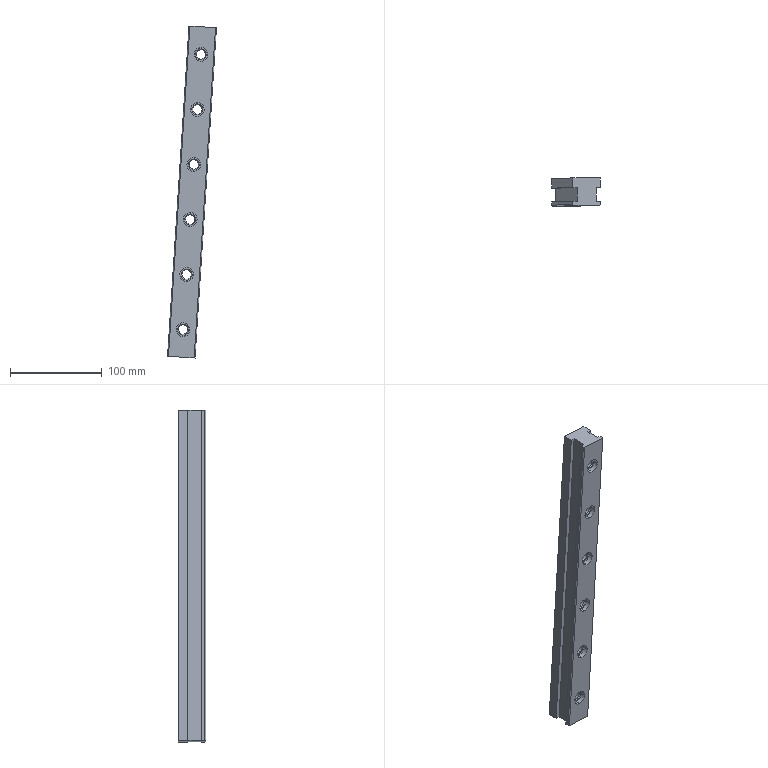Component | SolidWorks | GuideRail-4 | 1 solid | 58 faces | box 53.24 x 30 x 361.19 mm | volume 257394 mm3 | cylinder 24 | plane 22 | cone 12 | commonest cylinder face diameters 10.2 x12 15 x12
build123d program:
from build123d import *

# Parameters (mm, degrees)
SKETCH1_W                    = 360
SKETCH1_H                    = 30
BOSS_EXTRUDE1_DEPTH          = 30
CUT_EXTRUDE1_DEPTH           = 585.893
CUT_EXTRUDE1_DEPTH_BACK      = 585.893
SKETCH2_W                    = 15
SKETCH2_H                    = 9
SKETCH3_R                    = 7.5
CUT_EXTRUDE2_DEPTH           = 5
M12_TAPPED_HOLE1_D           = 10.2
M12_TAPPED_HOLE1_DEPTH       = 50
M12_TAPPED_HOLE1_CSINK_D     = 12.05
M12_TAPPED_HOLE1_CSINK_ANGLE = 90
M12_TAPPED_HOLE1_TIP         = 3.064
CHAMFER1_SIZE                = 1


with BuildPart() as part:
    # Sketch1 → Boss-Extrude1 (new body)
    with BuildSketch(Plane.XY):
        with Locations((-3.755, 445)):
            Rectangle(SKETCH1_W, SKETCH1_H)
    extrude(amount=BOSS_EXTRUDE1_DEPTH)

    # Sketch2 → Cut-Extrude1 (cut, two sides: drawn at the far end of the back side and taken through both)
    with BuildSketch(Plane.ZY.offset(183.755).offset(-CUT_EXTRUDE1_DEPTH_BACK)):
        with Locations((18, 460)):
            Rectangle(SKETCH2_W, SKETCH2_H)
        with Locations((18, 430)):
            Rectangle(SKETCH2_W, SKETCH2_H)
    extrude(amount=CUT_EXTRUDE1_DEPTH + CUT_EXTRUDE1_DEPTH_BACK, mode=Mode.SUBTRACT)

    # Sketch3 → Cut-Extrude2 (cut)
    with BuildSketch(Plane.XY.offset(30)):
        with Locations((146.245, 445)):
            Circle(SKETCH3_R)
        with Locations((86.245, 445)):
            Circle(SKETCH3_R)
        with Locations((26.245, 445)):
            Circle(SKETCH3_R)
        with Locations((-33.755, 445)):
            Circle(SKETCH3_R)
        with Locations((-93.755, 445)):
            Circle(SKETCH3_R)
        with Locations((-153.755, 445)):
            Circle(SKETCH3_R)
    extrude(amount=-CUT_EXTRUDE2_DEPTH, mode=Mode.SUBTRACT)

    # M12 Tapped Hole1
    with Locations(Plane(origin=(146.245, 445, 25), x_dir=(1, 0, 0), z_dir=(0, 0, 1))):
        with Locations((0, 0), (-60, 0), (-120, 0), (-180, 0), (-240, 0), (-300, 0)):
            CounterSinkHole(M12_TAPPED_HOLE1_D / 2, M12_TAPPED_HOLE1_CSINK_D / 2, depth=M12_TAPPED_HOLE1_DEPTH, counter_sink_angle=M12_TAPPED_HOLE1_CSINK_ANGLE)
            with Locations((0, 0, -(M12_TAPPED_HOLE1_DEPTH + M12_TAPPED_HOLE1_TIP / 2))):  # 118° drill point
                Cone(0, M12_TAPPED_HOLE1_D / 2, M12_TAPPED_HOLE1_TIP, mode=Mode.SUBTRACT)

    # Chamfer1
    chamfer1_edges = [part.edges().sort_by_distance(p)[0] for p in [
        (-3.755, 430, 30),
        (-3.755, 460, 30),
    ]]
    chamfer(chamfer1_edges, length=CHAMFER1_SIZE)


solid = part.part

# Placed as in the assembly
solid = solid.moved(Location((-304.927, -601, -288.99), (90, 0, -93.712)))